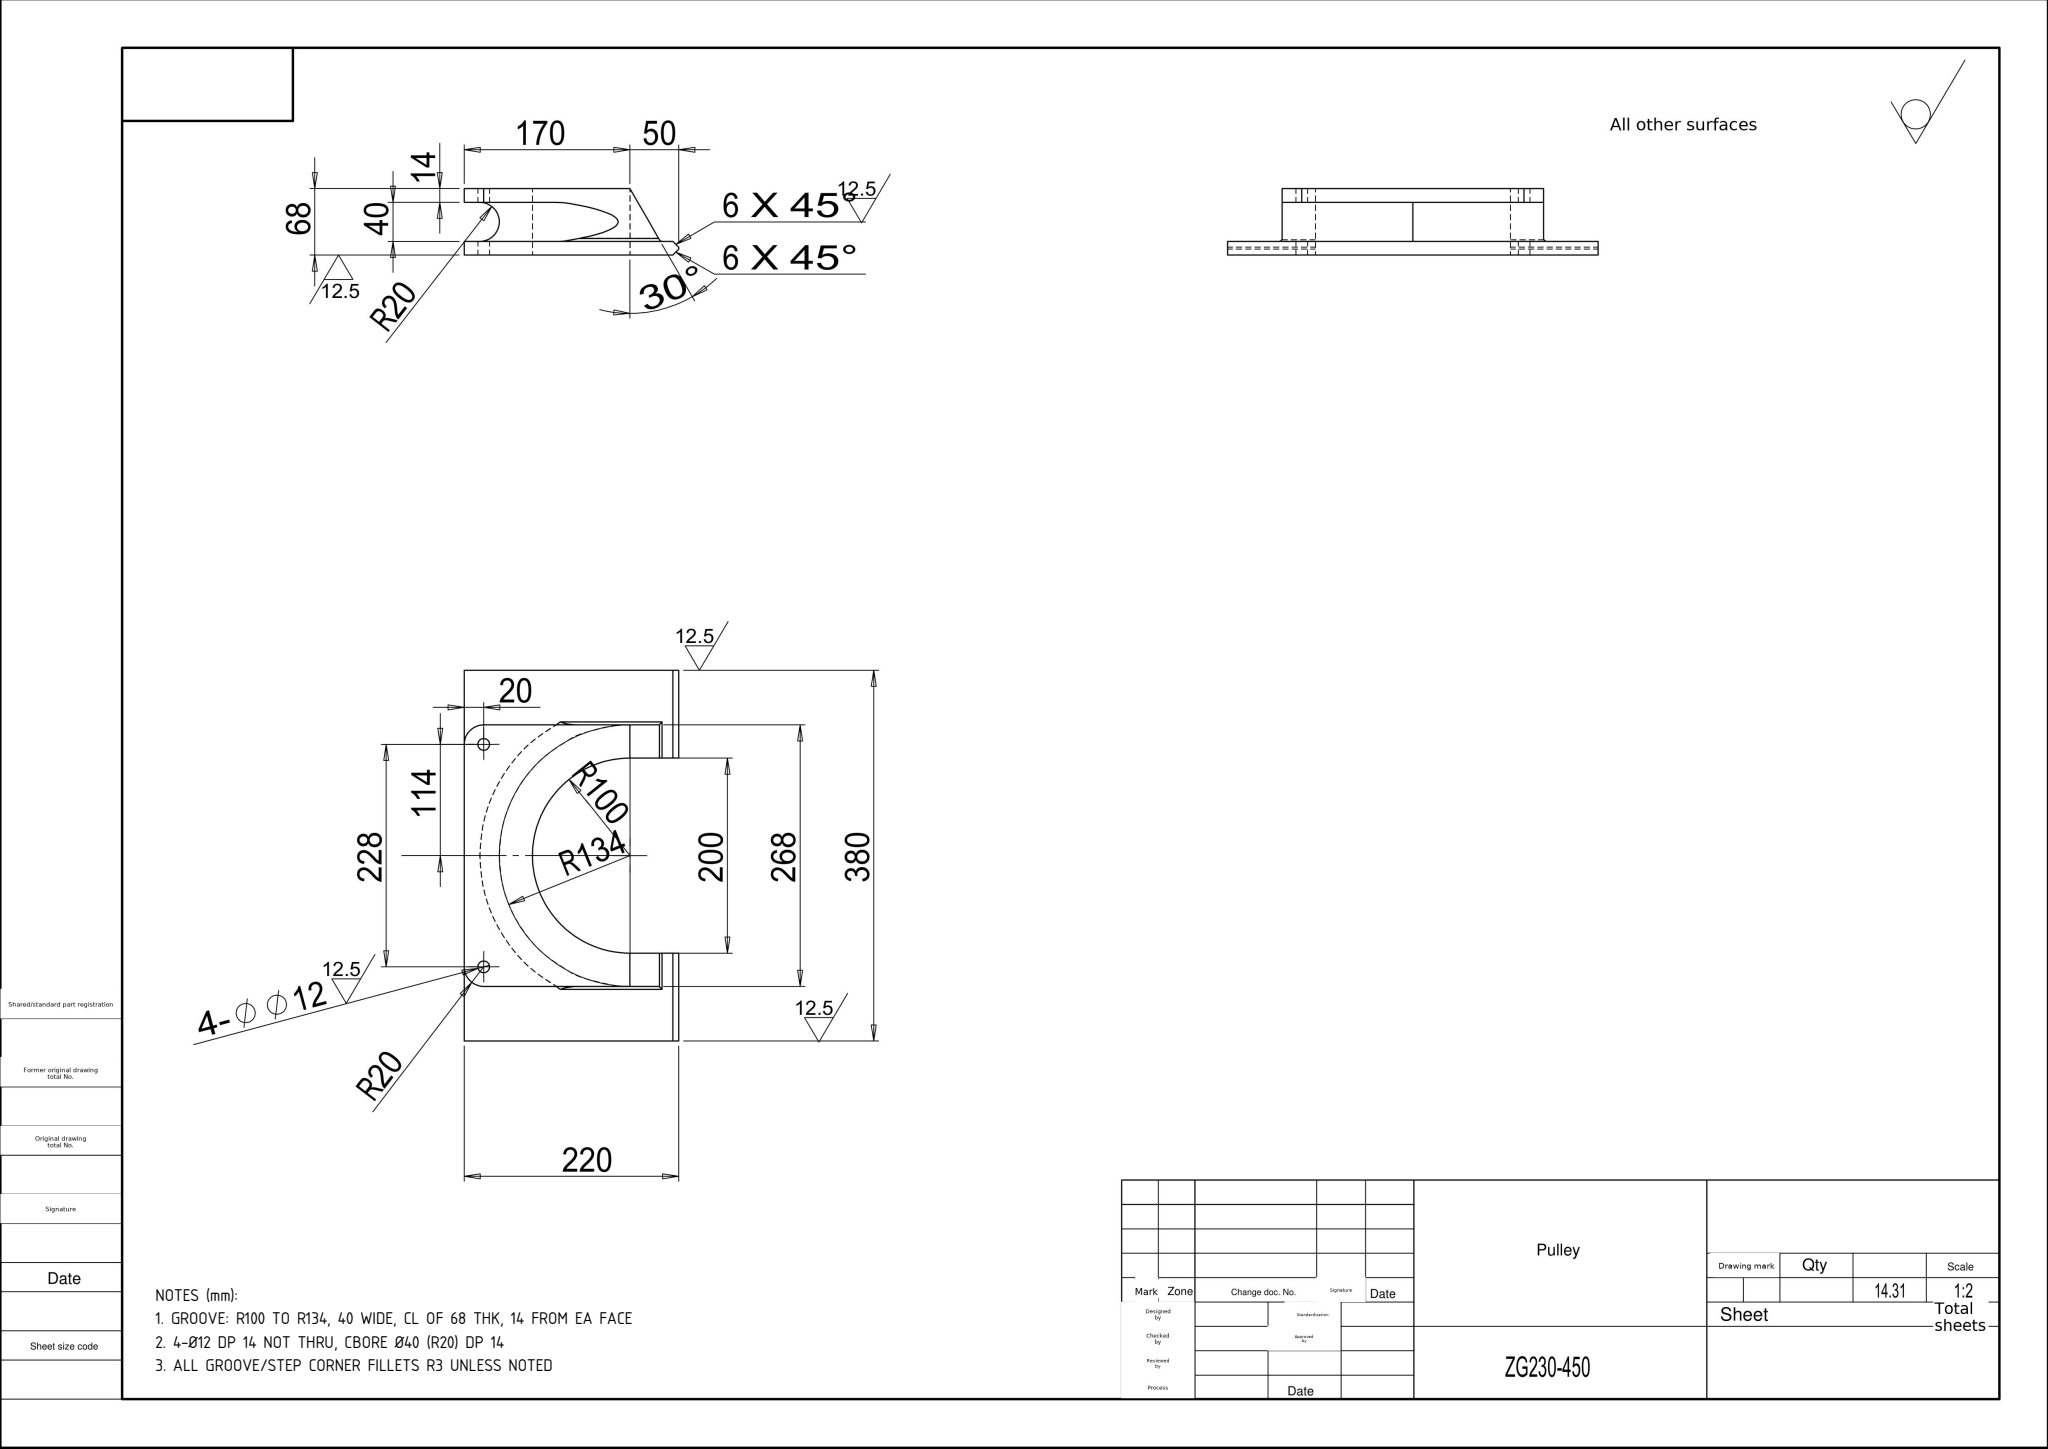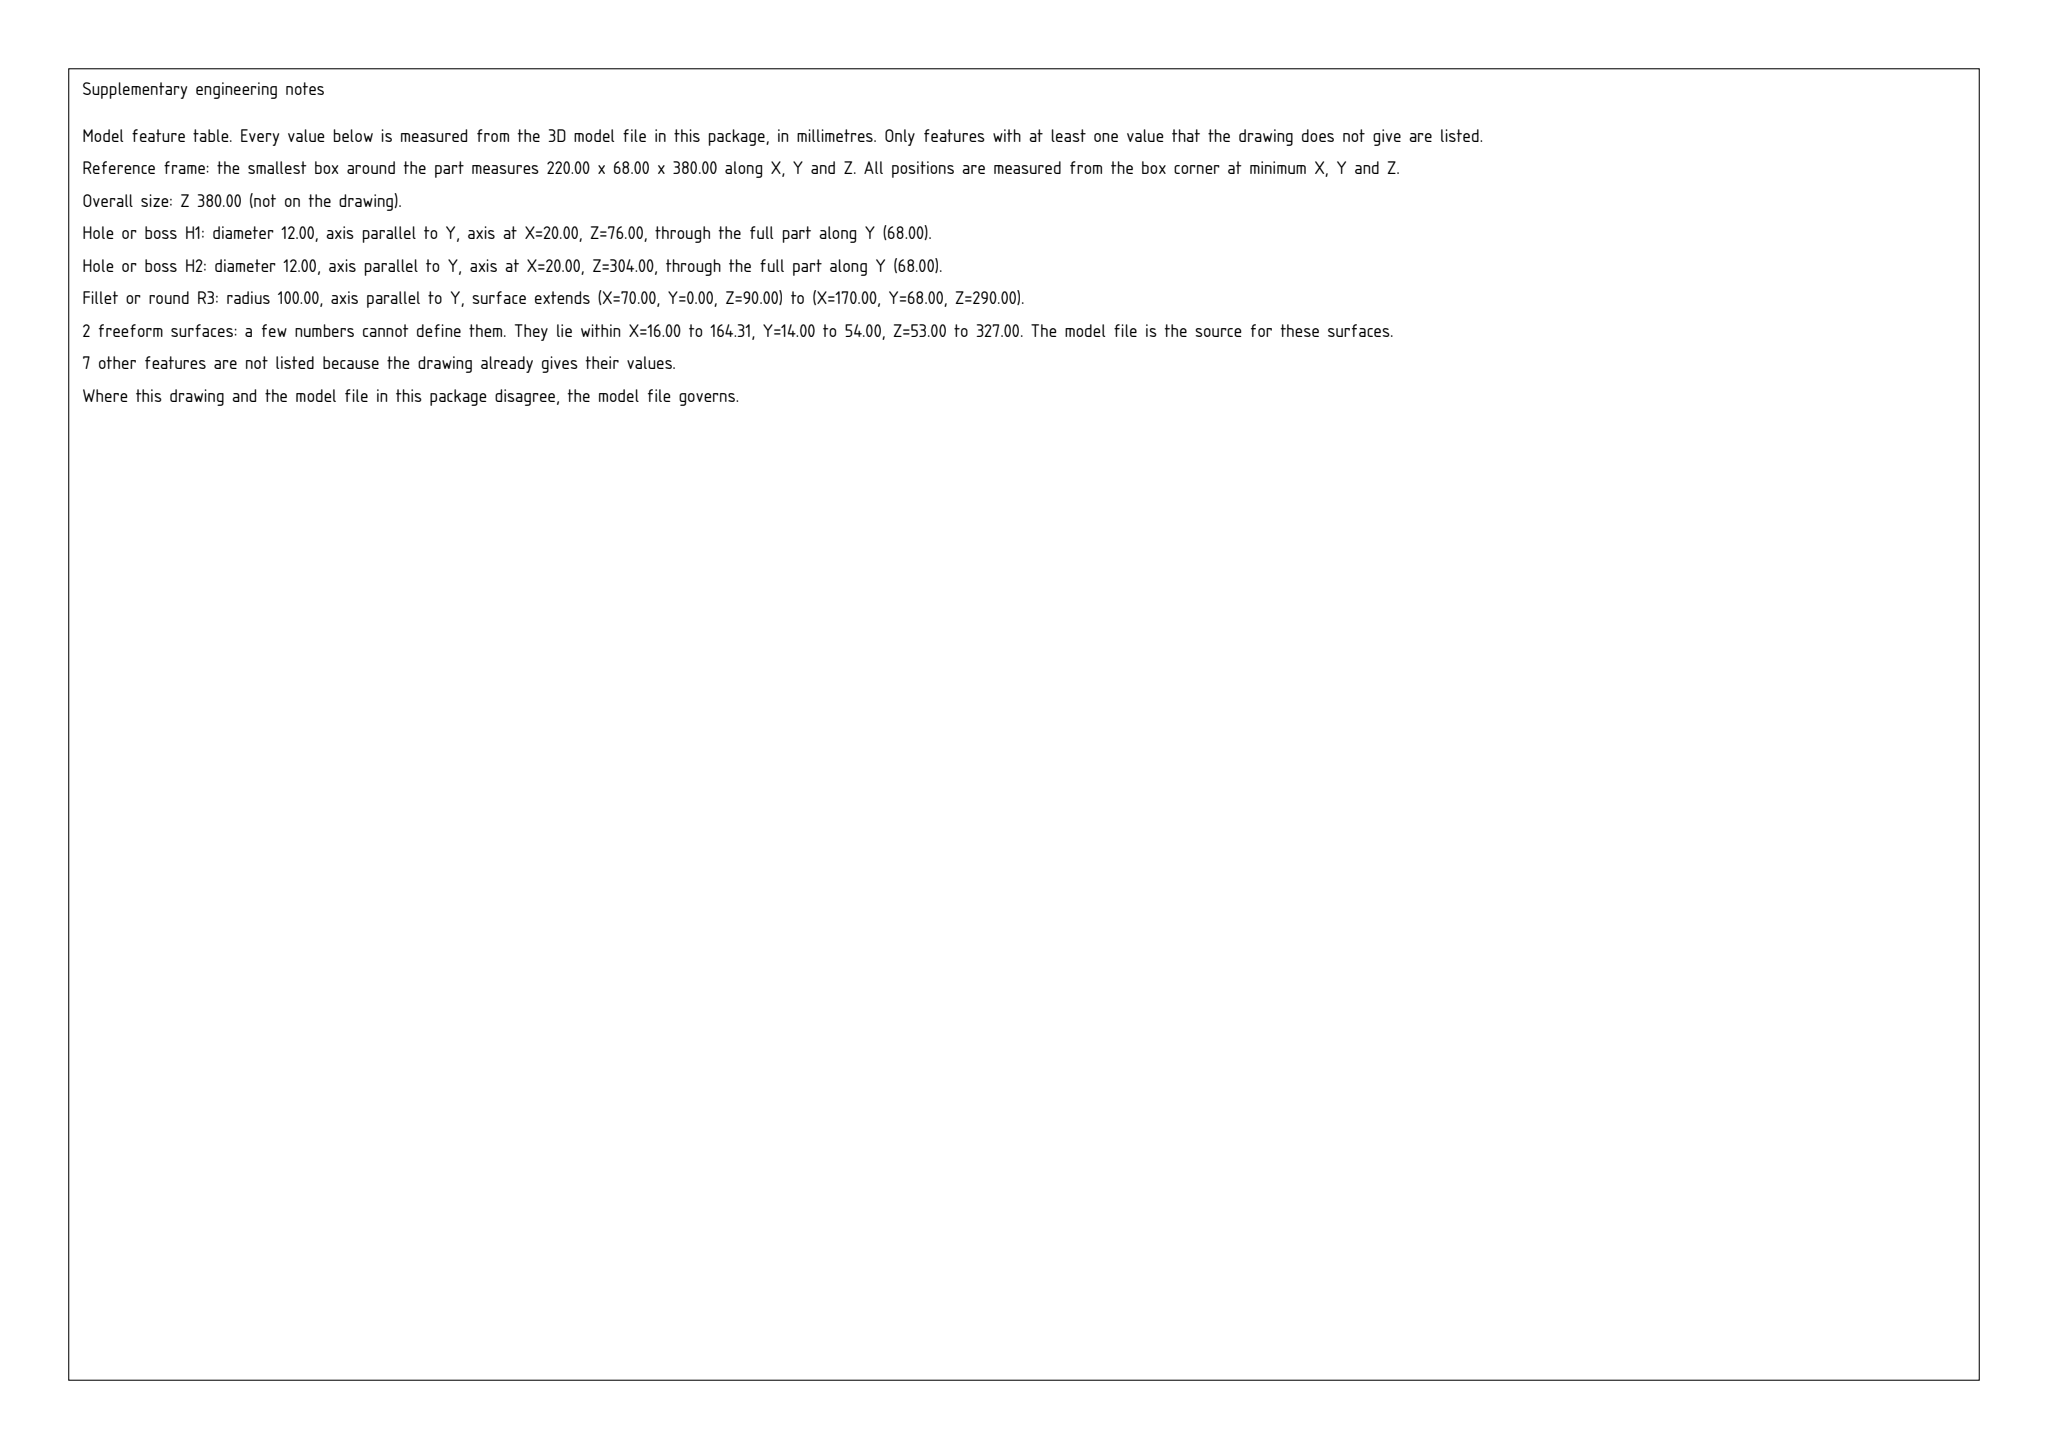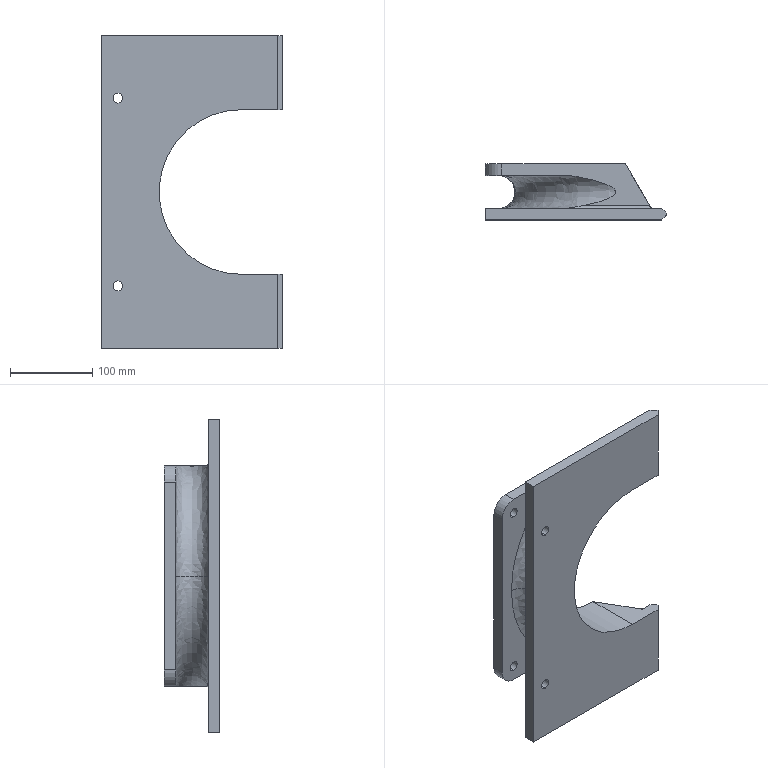Part | SolidWorks | mm | 1 solid | 37 faces | box 220 x 68 x 380 mm | volume 1834320 mm3 | plane 20 | cylinder 15 | spline 2 | commonest cylinder face diameters 12 x8 6 x4 40 x2 200 x1
Drawing notes:
GROOVE: R100 TO R134, 40 WIDE, CL OF 68 THK, 14 FROM EA FACE | from the solid: y-planes 0/14/54/68; Ø200 (R100) y-axis bore at x170,z190; R134 outer groove
4-Ø12 DP 14 NOT THRU, CBORE Ø40 (R20) DP 14 | from the solid: Ø12 y-axis cyls len 14 at (20,76)&(20,304); Ø40 y-axis cyls len 14 same centers
ALL GROOVE/STEP CORNER FILLETS R3 UNLESS NOTED | from the solid: Ø6 cyls (R3): x-axis at y17/z53 & z327; z-axis at x202.91,y17